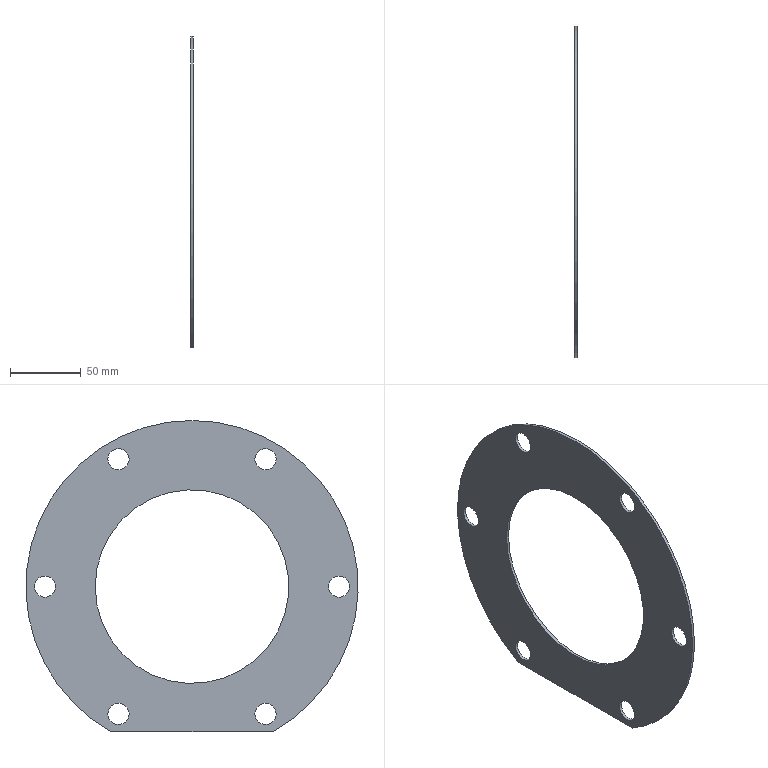Component | NX | T2_GASKET | 1 solid | 11 faces | box 2 x 235 x 220 mm | volume 52816 mm3 | cylinder 8 | plane 3 | commonest cylinder face diameters 15 x6 137 x1 235 x1
STEP:
#1=CARTESIAN_POINT('',(0.,0.,0.));
#2=DIRECTION('',(0.,0.,1.));
#3=DIRECTION('',(1.,0.,0.));
#4=AXIS2_PLACEMENT_3D('',#1,#2,#3);
#5=CARTESIAN_POINT('',(223.,-57.446,-105.5));
#6=VERTEX_POINT('',#5);
#7=CARTESIAN_POINT('',(223.,57.446,-105.5));
#8=VERTEX_POINT('',#7);
#9=CARTESIAN_POINT('',(223.,-57.446,-105.5));
#10=DIRECTION('',(0.,1.,0.));
#11=VECTOR('',#10,1.);
#12=LINE('',#9,#11);
#13=CARTESIAN_POINT('',(225.,-57.446,-105.5));
#14=DIRECTION('',(0.,0.,1.));
#15=DIRECTION('',(0.,1.,0.));
#16=AXIS2_PLACEMENT_3D('',#13,#14,#15);
#17=PLANE('',#16);
#18=CARTESIAN_POINT('',(0.,2.));
#19=DIRECTION('',(1.,0.));
#20=VECTOR('',#19,1.);
#21=LINE('',#18,#20);
#22=(GEOMETRIC_REPRESENTATION_CONTEXT(2)PARAMETRIC_REPRESENTATION_CONTEXT()REPRESENTATION_CONTEXT('',''));
#23=DEFINITIONAL_REPRESENTATION('',(#21),#22);
#24=PCURVE('',#17,#23);
#25=CARTESIAN_POINT('',(223.,0.,-3.));
#26=DIRECTION('',(1.,0.,0.));
#27=DIRECTION('',(0.,0.,-1.));
#28=AXIS2_PLACEMENT_3D('',#25,#26,#27);
#29=PLANE('',#28);
#30=CARTESIAN_POINT('',(102.5,-57.446));
#31=DIRECTION('',(0.,1.));
#32=VECTOR('',#31,1.);
#33=LINE('',#30,#32);
#34=(GEOMETRIC_REPRESENTATION_CONTEXT(2)PARAMETRIC_REPRESENTATION_CONTEXT()REPRESENTATION_CONTEXT('',''));
#35=DEFINITIONAL_REPRESENTATION('',(#33),#34);
#36=PCURVE('',#29,#35);
#37=SURFACE_CURVE('',#12,(#24,#36),.PCURVE_S1.);
#38=EDGE_CURVE('',#6,#8,#37,.T.);
#39=ORIENTED_EDGE('',*,*,#38,.T.);
#40=CARTESIAN_POINT('',(225.,57.446,-105.5));
#41=VERTEX_POINT('',#40);
#42=CARTESIAN_POINT('',(225.,57.446,-105.5));
#43=DIRECTION('',(-1.,0.,0.));
#44=VECTOR('',#43,1.);
#45=LINE('',#42,#44);
#46=CARTESIAN_POINT('',(114.891,0.));
#47=DIRECTION('',(0.,1.));
#48=VECTOR('',#47,1.);
#49=LINE('',#46,#48);
#50=(GEOMETRIC_REPRESENTATION_CONTEXT(2)PARAMETRIC_REPRESENTATION_CONTEXT()REPRESENTATION_CONTEXT('',''));
#51=DEFINITIONAL_REPRESENTATION('',(#49),#50);
#52=PCURVE('',#17,#51);
#53=CARTESIAN_POINT('',(225.,0.,-3.));
#54=DIRECTION('',(-1.,0.,0.));
#55=DIRECTION('',(0.,0.,1.));
#56=AXIS2_PLACEMENT_3D('',#53,#54,#55);
#57=CYLINDRICAL_SURFACE('',#56,117.5);
#58=CARTESIAN_POINT('',(2.631,0.));
#59=DIRECTION('',(0.,1.));
#60=VECTOR('',#59,1.);
#61=LINE('',#58,#60);
#62=(GEOMETRIC_REPRESENTATION_CONTEXT(2)PARAMETRIC_REPRESENTATION_CONTEXT()REPRESENTATION_CONTEXT('',''));
#63=DEFINITIONAL_REPRESENTATION('',(#61),#62);
#64=PCURVE('',#57,#63);
#65=SURFACE_CURVE('',#45,(#52,#64),.PCURVE_S1.);
#66=EDGE_CURVE('',#41,#8,#65,.T.);
#67=ORIENTED_EDGE('',*,*,#66,.F.);
#68=CARTESIAN_POINT('',(225.,-57.446,-105.5));
#69=VERTEX_POINT('',#68);
#70=CARTESIAN_POINT('',(225.,-57.446,-105.5));
#71=DIRECTION('',(0.,1.,0.));
#72=VECTOR('',#71,1.);
#73=LINE('',#70,#72);
#74=CARTESIAN_POINT('',(0.,0.));
#75=DIRECTION('',(1.,0.));
#76=VECTOR('',#75,1.);
#77=LINE('',#74,#76);
#78=(GEOMETRIC_REPRESENTATION_CONTEXT(2)PARAMETRIC_REPRESENTATION_CONTEXT()REPRESENTATION_CONTEXT('',''));
#79=DEFINITIONAL_REPRESENTATION('',(#77),#78);
#80=PCURVE('',#17,#79);
#81=CARTESIAN_POINT('',(225.,0.,-3.));
#82=DIRECTION('',(1.,0.,0.));
#83=DIRECTION('',(0.,0.,-1.));
#84=AXIS2_PLACEMENT_3D('',#81,#82,#83);
#85=PLANE('',#84);
#86=CARTESIAN_POINT('',(102.5,-57.446));
#87=DIRECTION('',(0.,1.));
#88=VECTOR('',#87,1.);
#89=LINE('',#86,#88);
#90=(GEOMETRIC_REPRESENTATION_CONTEXT(2)PARAMETRIC_REPRESENTATION_CONTEXT()REPRESENTATION_CONTEXT('',''));
#91=DEFINITIONAL_REPRESENTATION('',(#89),#90);
#92=PCURVE('',#85,#91);
#93=SURFACE_CURVE('',#73,(#80,#92),.PCURVE_S1.);
#94=EDGE_CURVE('',#69,#41,#93,.T.);
#95=ORIENTED_EDGE('',*,*,#94,.F.);
#96=CARTESIAN_POINT('',(225.,-57.446,-105.5));
#97=DIRECTION('',(1.,0.,0.));
#98=VECTOR('',#97,1.);
#99=LINE('',#96,#98);
#100=CARTESIAN_POINT('',(0.,0.));
#101=DIRECTION('',(0.,-1.));
#102=VECTOR('',#101,1.);
#103=LINE('',#100,#102);
#104=(GEOMETRIC_REPRESENTATION_CONTEXT(2)PARAMETRIC_REPRESENTATION_CONTEXT()REPRESENTATION_CONTEXT('',''));
#105=DEFINITIONAL_REPRESENTATION('',(#103),#104);
#106=PCURVE('',#17,#105);
#107=CARTESIAN_POINT('',(-2.631,0.));
#108=DIRECTION('',(0.,-1.));
#109=VECTOR('',#108,1.);
#110=LINE('',#107,#109);
#111=(GEOMETRIC_REPRESENTATION_CONTEXT(2)PARAMETRIC_REPRESENTATION_CONTEXT()REPRESENTATION_CONTEXT('',''));
#112=DEFINITIONAL_REPRESENTATION('',(#110),#111);
#113=PCURVE('',#57,#112);
#114=SURFACE_CURVE('',#99,(#106,#113),.PCURVE_S1.);
#115=EDGE_CURVE('',#6,#69,#114,.T.);
#116=ORIENTED_EDGE('',*,*,#115,.F.);
#117=EDGE_LOOP('',(#39,#67,#95,#116));
#118=FACE_BOUND('',#117,.T.);
#119=ADVANCED_FACE('',(#118),#17,.F.);
#120=CARTESIAN_POINT('',(225.,55.75,-99.562));
#121=VERTEX_POINT('',#120);
#122=CARTESIAN_POINT('',(225.,52.,-93.067));
#123=DIRECTION('',(1.,0.,0.));
#124=DIRECTION('',(0.,0.5,-0.866));
#125=AXIS2_PLACEMENT_3D('',#122,#123,#124);
#126=CIRCLE('',#125,7.5);
#127=CARTESIAN_POINT('',(225.,52.,-93.067));
#128=DIRECTION('',(-1.,0.,0.));
#129=DIRECTION('',(0.,0.,1.));
#130=AXIS2_PLACEMENT_3D('',#127,#128,#129);
#131=CYLINDRICAL_SURFACE('',#130,7.5);
#132=CARTESIAN_POINT('',(8.901,0.));
#133=DIRECTION('',(-1.,0.));
#134=VECTOR('',#133,1.);
#135=LINE('',#132,#134);
#136=(GEOMETRIC_REPRESENTATION_CONTEXT(2)PARAMETRIC_REPRESENTATION_CONTEXT()REPRESENTATION_CONTEXT('',''));
#137=DEFINITIONAL_REPRESENTATION('',(#135),#136);
#138=PCURVE('',#131,#137);
#139=CARTESIAN_POINT('',(90.067,52.));
#140=DIRECTION('',(0.866,0.5));
#141=AXIS2_PLACEMENT_2D('',#139,#140);
#142=CIRCLE('',#141,7.5);
#143=(GEOMETRIC_REPRESENTATION_CONTEXT(2)PARAMETRIC_REPRESENTATION_CONTEXT()REPRESENTATION_CONTEXT('',''));
#144=DEFINITIONAL_REPRESENTATION('',(#142),#143);
#145=PCURVE('',#85,#144);
#146=SURFACE_CURVE('',#126,(#138,#145),.PCURVE_S1.);
#147=EDGE_CURVE('',#121,#121,#146,.T.);
#148=ORIENTED_EDGE('',*,*,#147,.F.);
#149=CARTESIAN_POINT('',(223.,55.75,-99.562));
#150=VERTEX_POINT('',#149);
#151=CARTESIAN_POINT('',(225.,55.75,-99.562));
#152=CARTESIAN_POINT('',(223.,55.75,-99.562));
#153=B_SPLINE_CURVE_WITH_KNOTS('',1,(#151,#152),.UNSPECIFIED.,.F.,.F.,(2,2),(0.,2.),.PIECEWISE_BEZIER_KNOTS.);
#154=CARTESIAN_POINT('',(8.901,0.));
#155=DIRECTION('',(0.,1.));
#156=VECTOR('',#155,1.);
#157=LINE('',#154,#156);
#158=(GEOMETRIC_REPRESENTATION_CONTEXT(2)PARAMETRIC_REPRESENTATION_CONTEXT()REPRESENTATION_CONTEXT('',''));
#159=DEFINITIONAL_REPRESENTATION('',(#157),#158);
#160=PCURVE('',#131,#159);
#161=CARTESIAN_POINT('',(2.618,0.));
#162=DIRECTION('',(0.,1.));
#163=VECTOR('',#162,1.);
#164=LINE('',#161,#163);
#165=(GEOMETRIC_REPRESENTATION_CONTEXT(2)PARAMETRIC_REPRESENTATION_CONTEXT()REPRESENTATION_CONTEXT('',''));
#166=DEFINITIONAL_REPRESENTATION('',(#164),#165);
#167=PCURVE('',#131,#166);
#168=SEAM_CURVE('',#153,(#160,#167),.PCURVE_S1.);
#169=EDGE_CURVE('',#121,#150,#168,.T.);
#170=ORIENTED_EDGE('',*,*,#169,.T.);
#171=CARTESIAN_POINT('',(223.,52.,-93.067));
#172=DIRECTION('',(1.,0.,0.));
#173=DIRECTION('',(0.,0.5,-0.866));
#174=AXIS2_PLACEMENT_3D('',#171,#172,#173);
#175=CIRCLE('',#174,7.5);
#176=CARTESIAN_POINT('',(8.901,2.));
#177=DIRECTION('',(-1.,0.));
#178=VECTOR('',#177,1.);
#179=LINE('',#176,#178);
#180=(GEOMETRIC_REPRESENTATION_CONTEXT(2)PARAMETRIC_REPRESENTATION_CONTEXT()REPRESENTATION_CONTEXT('',''));
#181=DEFINITIONAL_REPRESENTATION('',(#179),#180);
#182=PCURVE('',#131,#181);
#183=CARTESIAN_POINT('',(90.067,52.));
#184=DIRECTION('',(0.866,0.5));
#185=AXIS2_PLACEMENT_2D('',#183,#184);
#186=CIRCLE('',#185,7.5);
#187=(GEOMETRIC_REPRESENTATION_CONTEXT(2)PARAMETRIC_REPRESENTATION_CONTEXT()REPRESENTATION_CONTEXT('',''));
#188=DEFINITIONAL_REPRESENTATION('',(#186),#187);
#189=PCURVE('',#29,#188);
#190=SURFACE_CURVE('',#175,(#182,#189),.PCURVE_S1.);
#191=EDGE_CURVE('',#150,#150,#190,.T.);
#192=ORIENTED_EDGE('',*,*,#191,.T.);
#193=ORIENTED_EDGE('',*,*,#169,.F.);
#194=EDGE_LOOP('',(#148,#170,#192,#193));
#195=FACE_BOUND('',#194,.F.);
#196=ADVANCED_FACE('',(#195),#131,.F.);
#197=CARTESIAN_POINT('',(225.,-55.75,-99.562));
#198=VERTEX_POINT('',#197);
#199=CARTESIAN_POINT('',(225.,-52.,-93.067));
#200=DIRECTION('',(1.,0.,0.));
#201=DIRECTION('',(0.,-0.5,-0.866));
#202=AXIS2_PLACEMENT_3D('',#199,#200,#201);
#203=CIRCLE('',#202,7.5);
#204=CARTESIAN_POINT('',(225.,-52.,-93.067));
#205=DIRECTION('',(-1.,0.,0.));
#206=DIRECTION('',(0.,0.,1.));
#207=AXIS2_PLACEMENT_3D('',#204,#205,#206);
#208=CYLINDRICAL_SURFACE('',#207,7.5);
#209=CARTESIAN_POINT('',(9.948,0.));
#210=DIRECTION('',(-1.,0.));
#211=VECTOR('',#210,1.);
#212=LINE('',#209,#211);
#213=(GEOMETRIC_REPRESENTATION_CONTEXT(2)PARAMETRIC_REPRESENTATION_CONTEXT()REPRESENTATION_CONTEXT('',''));
#214=DEFINITIONAL_REPRESENTATION('',(#212),#213);
#215=PCURVE('',#208,#214);
#216=CARTESIAN_POINT('',(90.067,-52.));
#217=DIRECTION('',(0.866,-0.5));
#218=AXIS2_PLACEMENT_2D('',#216,#217);
#219=CIRCLE('',#218,7.5);
#220=(GEOMETRIC_REPRESENTATION_CONTEXT(2)PARAMETRIC_REPRESENTATION_CONTEXT()REPRESENTATION_CONTEXT('',''));
#221=DEFINITIONAL_REPRESENTATION('',(#219),#220);
#222=PCURVE('',#85,#221);
#223=SURFACE_CURVE('',#203,(#215,#222),.PCURVE_S1.);
#224=EDGE_CURVE('',#198,#198,#223,.T.);
#225=ORIENTED_EDGE('',*,*,#224,.F.);
#226=CARTESIAN_POINT('',(223.,-55.75,-99.562));
#227=VERTEX_POINT('',#226);
#228=CARTESIAN_POINT('',(225.,-55.75,-99.562));
#229=CARTESIAN_POINT('',(223.,-55.75,-99.562));
#230=B_SPLINE_CURVE_WITH_KNOTS('',1,(#228,#229),.UNSPECIFIED.,.F.,.F.,(2,2),(0.,2.),.PIECEWISE_BEZIER_KNOTS.);
#231=CARTESIAN_POINT('',(9.948,0.));
#232=DIRECTION('',(0.,1.));
#233=VECTOR('',#232,1.);
#234=LINE('',#231,#233);
#235=(GEOMETRIC_REPRESENTATION_CONTEXT(2)PARAMETRIC_REPRESENTATION_CONTEXT()REPRESENTATION_CONTEXT('',''));
#236=DEFINITIONAL_REPRESENTATION('',(#234),#235);
#237=PCURVE('',#208,#236);
#238=CARTESIAN_POINT('',(3.665,0.));
#239=DIRECTION('',(0.,1.));
#240=VECTOR('',#239,1.);
#241=LINE('',#238,#240);
#242=(GEOMETRIC_REPRESENTATION_CONTEXT(2)PARAMETRIC_REPRESENTATION_CONTEXT()REPRESENTATION_CONTEXT('',''));
#243=DEFINITIONAL_REPRESENTATION('',(#241),#242);
#244=PCURVE('',#208,#243);
#245=SEAM_CURVE('',#230,(#237,#244),.PCURVE_S1.);
#246=EDGE_CURVE('',#198,#227,#245,.T.);
#247=ORIENTED_EDGE('',*,*,#246,.T.);
#248=CARTESIAN_POINT('',(223.,-52.,-93.067));
#249=DIRECTION('',(1.,0.,0.));
#250=DIRECTION('',(0.,-0.5,-0.866));
#251=AXIS2_PLACEMENT_3D('',#248,#249,#250);
#252=CIRCLE('',#251,7.5);
#253=CARTESIAN_POINT('',(9.948,2.));
#254=DIRECTION('',(-1.,0.));
#255=VECTOR('',#254,1.);
#256=LINE('',#253,#255);
#257=(GEOMETRIC_REPRESENTATION_CONTEXT(2)PARAMETRIC_REPRESENTATION_CONTEXT()REPRESENTATION_CONTEXT('',''));
#258=DEFINITIONAL_REPRESENTATION('',(#256),#257);
#259=PCURVE('',#208,#258);
#260=CARTESIAN_POINT('',(90.067,-52.));
#261=DIRECTION('',(0.866,-0.5));
#262=AXIS2_PLACEMENT_2D('',#260,#261);
#263=CIRCLE('',#262,7.5);
#264=(GEOMETRIC_REPRESENTATION_CONTEXT(2)PARAMETRIC_REPRESENTATION_CONTEXT()REPRESENTATION_CONTEXT('',''));
#265=DEFINITIONAL_REPRESENTATION('',(#263),#264);
#266=PCURVE('',#29,#265);
#267=SURFACE_CURVE('',#252,(#259,#266),.PCURVE_S1.);
#268=EDGE_CURVE('',#227,#227,#267,.T.);
#269=ORIENTED_EDGE('',*,*,#268,.T.);
#270=ORIENTED_EDGE('',*,*,#246,.F.);
#271=EDGE_LOOP('',(#225,#247,#269,#270));
#272=FACE_BOUND('',#271,.F.);
#273=ADVANCED_FACE('',(#272),#208,.F.);
#274=CARTESIAN_POINT('',(225.,-111.5,-3.));
#275=VERTEX_POINT('',#274);
#276=CARTESIAN_POINT('',(225.,-104.,-3.));
#277=DIRECTION('',(1.,0.,0.));
#278=DIRECTION('',(0.,-1.,0.));
#279=AXIS2_PLACEMENT_3D('',#276,#277,#278);
#280=CIRCLE('',#279,7.5);
#281=CARTESIAN_POINT('',(225.,-104.,-3.));
#282=DIRECTION('',(-1.,0.,0.));
#283=DIRECTION('',(0.,0.,1.));
#284=AXIS2_PLACEMENT_3D('',#281,#282,#283);
#285=CYLINDRICAL_SURFACE('',#284,7.5);
#286=CARTESIAN_POINT('',(10.996,0.));
#287=DIRECTION('',(-1.,0.));
#288=VECTOR('',#287,1.);
#289=LINE('',#286,#288);
#290=(GEOMETRIC_REPRESENTATION_CONTEXT(2)PARAMETRIC_REPRESENTATION_CONTEXT()REPRESENTATION_CONTEXT('',''));
#291=DEFINITIONAL_REPRESENTATION('',(#289),#290);
#292=PCURVE('',#285,#291);
#293=CARTESIAN_POINT('',(0.,-104.));
#294=DIRECTION('',(-0.,-1.));
#295=AXIS2_PLACEMENT_2D('',#293,#294);
#296=CIRCLE('',#295,7.5);
#297=(GEOMETRIC_REPRESENTATION_CONTEXT(2)PARAMETRIC_REPRESENTATION_CONTEXT()REPRESENTATION_CONTEXT('',''));
#298=DEFINITIONAL_REPRESENTATION('',(#296),#297);
#299=PCURVE('',#85,#298);
#300=SURFACE_CURVE('',#280,(#292,#299),.PCURVE_S1.);
#301=EDGE_CURVE('',#275,#275,#300,.T.);
#302=ORIENTED_EDGE('',*,*,#301,.F.);
#303=CARTESIAN_POINT('',(223.,-111.5,-3.));
#304=VERTEX_POINT('',#303);
#305=CARTESIAN_POINT('',(225.,-111.5,-3.));
#306=CARTESIAN_POINT('',(223.,-111.5,-3.));
#307=B_SPLINE_CURVE_WITH_KNOTS('',1,(#305,#306),.UNSPECIFIED.,.F.,.F.,(2,2),(0.,2.),.PIECEWISE_BEZIER_KNOTS.);
#308=CARTESIAN_POINT('',(10.996,0.));
#309=DIRECTION('',(0.,1.));
#310=VECTOR('',#309,1.);
#311=LINE('',#308,#310);
#312=(GEOMETRIC_REPRESENTATION_CONTEXT(2)PARAMETRIC_REPRESENTATION_CONTEXT()REPRESENTATION_CONTEXT('',''));
#313=DEFINITIONAL_REPRESENTATION('',(#311),#312);
#314=PCURVE('',#285,#313);
#315=CARTESIAN_POINT('',(4.712,0.));
#316=DIRECTION('',(0.,1.));
#317=VECTOR('',#316,1.);
#318=LINE('',#315,#317);
#319=(GEOMETRIC_REPRESENTATION_CONTEXT(2)PARAMETRIC_REPRESENTATION_CONTEXT()REPRESENTATION_CONTEXT('',''));
#320=DEFINITIONAL_REPRESENTATION('',(#318),#319);
#321=PCURVE('',#285,#320);
#322=SEAM_CURVE('',#307,(#314,#321),.PCURVE_S1.);
#323=EDGE_CURVE('',#275,#304,#322,.T.);
#324=ORIENTED_EDGE('',*,*,#323,.T.);
#325=CARTESIAN_POINT('',(223.,-104.,-3.));
#326=DIRECTION('',(1.,0.,0.));
#327=DIRECTION('',(0.,-1.,0.));
#328=AXIS2_PLACEMENT_3D('',#325,#326,#327);
#329=CIRCLE('',#328,7.5);
#330=CARTESIAN_POINT('',(10.996,2.));
#331=DIRECTION('',(-1.,0.));
#332=VECTOR('',#331,1.);
#333=LINE('',#330,#332);
#334=(GEOMETRIC_REPRESENTATION_CONTEXT(2)PARAMETRIC_REPRESENTATION_CONTEXT()REPRESENTATION_CONTEXT('',''));
#335=DEFINITIONAL_REPRESENTATION('',(#333),#334);
#336=PCURVE('',#285,#335);
#337=CARTESIAN_POINT('',(0.,-104.));
#338=DIRECTION('',(-0.,-1.));
#339=AXIS2_PLACEMENT_2D('',#337,#338);
#340=CIRCLE('',#339,7.5);
#341=(GEOMETRIC_REPRESENTATION_CONTEXT(2)PARAMETRIC_REPRESENTATION_CONTEXT()REPRESENTATION_CONTEXT('',''));
#342=DEFINITIONAL_REPRESENTATION('',(#340),#341);
#343=PCURVE('',#29,#342);
#344=SURFACE_CURVE('',#329,(#336,#343),.PCURVE_S1.);
#345=EDGE_CURVE('',#304,#304,#344,.T.);
#346=ORIENTED_EDGE('',*,*,#345,.T.);
#347=ORIENTED_EDGE('',*,*,#323,.F.);
#348=EDGE_LOOP('',(#302,#324,#346,#347));
#349=FACE_BOUND('',#348,.F.);
#350=ADVANCED_FACE('',(#349),#285,.F.);
#351=CARTESIAN_POINT('',(225.,68.5,-3.));
#352=VERTEX_POINT('',#351);
#353=CARTESIAN_POINT('',(225.,0.,-3.));
#354=DIRECTION('',(1.,0.,0.));
#355=DIRECTION('',(0.,1.,-0.));
#356=AXIS2_PLACEMENT_3D('',#353,#354,#355);
#357=CIRCLE('',#356,68.5);
#358=CARTESIAN_POINT('',(225.,0.,-3.));
#359=DIRECTION('',(-1.,0.,0.));
#360=DIRECTION('',(0.,0.,1.));
#361=AXIS2_PLACEMENT_3D('',#358,#359,#360);
#362=CYLINDRICAL_SURFACE('',#361,68.5);
#363=CARTESIAN_POINT('',(7.854,0.));
#364=DIRECTION('',(-1.,0.));
#365=VECTOR('',#364,1.);
#366=LINE('',#363,#365);
#367=(GEOMETRIC_REPRESENTATION_CONTEXT(2)PARAMETRIC_REPRESENTATION_CONTEXT()REPRESENTATION_CONTEXT('',''));
#368=DEFINITIONAL_REPRESENTATION('',(#366),#367);
#369=PCURVE('',#362,#368);
#370=CARTESIAN_POINT('',(0.,0.));
#371=DIRECTION('',(0.,1.));
#372=AXIS2_PLACEMENT_2D('',#370,#371);
#373=CIRCLE('',#372,68.5);
#374=(GEOMETRIC_REPRESENTATION_CONTEXT(2)PARAMETRIC_REPRESENTATION_CONTEXT()REPRESENTATION_CONTEXT('',''));
#375=DEFINITIONAL_REPRESENTATION('',(#373),#374);
#376=PCURVE('',#85,#375);
#377=SURFACE_CURVE('',#357,(#369,#376),.PCURVE_S1.);
#378=EDGE_CURVE('',#352,#352,#377,.T.);
#379=ORIENTED_EDGE('',*,*,#378,.F.);
#380=CARTESIAN_POINT('',(223.,68.5,-3.));
#381=VERTEX_POINT('',#380);
#382=CARTESIAN_POINT('',(225.,68.5,-3.));
#383=CARTESIAN_POINT('',(223.,68.5,-3.));
#384=B_SPLINE_CURVE_WITH_KNOTS('',1,(#382,#383),.UNSPECIFIED.,.F.,.F.,(2,2),(0.,2.),.PIECEWISE_BEZIER_KNOTS.);
#385=CARTESIAN_POINT('',(7.854,0.));
#386=DIRECTION('',(0.,1.));
#387=VECTOR('',#386,1.);
#388=LINE('',#385,#387);
#389=(GEOMETRIC_REPRESENTATION_CONTEXT(2)PARAMETRIC_REPRESENTATION_CONTEXT()REPRESENTATION_CONTEXT('',''));
#390=DEFINITIONAL_REPRESENTATION('',(#388),#389);
#391=PCURVE('',#362,#390);
#392=CARTESIAN_POINT('',(1.571,0.));
#393=DIRECTION('',(0.,1.));
#394=VECTOR('',#393,1.);
#395=LINE('',#392,#394);
#396=(GEOMETRIC_REPRESENTATION_CONTEXT(2)PARAMETRIC_REPRESENTATION_CONTEXT()REPRESENTATION_CONTEXT('',''));
#397=DEFINITIONAL_REPRESENTATION('',(#395),#396);
#398=PCURVE('',#362,#397);
#399=SEAM_CURVE('',#384,(#391,#398),.PCURVE_S1.);
#400=EDGE_CURVE('',#352,#381,#399,.T.);
#401=ORIENTED_EDGE('',*,*,#400,.T.);
#402=CARTESIAN_POINT('',(223.,0.,-3.));
#403=DIRECTION('',(1.,0.,0.));
#404=DIRECTION('',(0.,1.,-0.));
#405=AXIS2_PLACEMENT_3D('',#402,#403,#404);
#406=CIRCLE('',#405,68.5);
#407=CARTESIAN_POINT('',(7.854,2.));
#408=DIRECTION('',(-1.,0.));
#409=VECTOR('',#408,1.);
#410=LINE('',#407,#409);
#411=(GEOMETRIC_REPRESENTATION_CONTEXT(2)PARAMETRIC_REPRESENTATION_CONTEXT()REPRESENTATION_CONTEXT('',''));
#412=DEFINITIONAL_REPRESENTATION('',(#410),#411);
#413=PCURVE('',#362,#412);
#414=CARTESIAN_POINT('',(0.,0.));
#415=DIRECTION('',(0.,1.));
#416=AXIS2_PLACEMENT_2D('',#414,#415);
#417=CIRCLE('',#416,68.5);
#418=(GEOMETRIC_REPRESENTATION_CONTEXT(2)PARAMETRIC_REPRESENTATION_CONTEXT()REPRESENTATION_CONTEXT('',''));
#419=DEFINITIONAL_REPRESENTATION('',(#417),#418);
#420=PCURVE('',#29,#419);
#421=SURFACE_CURVE('',#406,(#413,#420),.PCURVE_S1.);
#422=EDGE_CURVE('',#381,#381,#421,.T.);
#423=ORIENTED_EDGE('',*,*,#422,.T.);
#424=ORIENTED_EDGE('',*,*,#400,.F.);
#425=EDGE_LOOP('',(#379,#401,#423,#424));
#426=FACE_BOUND('',#425,.F.);
#427=ADVANCED_FACE('',(#426),#362,.F.);
#428=CARTESIAN_POINT('',(225.,-55.75,93.562));
#429=VERTEX_POINT('',#428);
#430=CARTESIAN_POINT('',(225.,-52.,87.067));
#431=DIRECTION('',(1.,0.,0.));
#432=DIRECTION('',(0.,-0.5,0.866));
#433=AXIS2_PLACEMENT_3D('',#430,#431,#432);
#434=CIRCLE('',#433,7.5);
#435=CARTESIAN_POINT('',(225.,-52.,87.067));
#436=DIRECTION('',(-1.,0.,0.));
#437=DIRECTION('',(0.,0.,1.));
#438=AXIS2_PLACEMENT_3D('',#435,#436,#437);
#439=CYLINDRICAL_SURFACE('',#438,7.5);
#440=CARTESIAN_POINT('',(12.043,0.));
#441=DIRECTION('',(-1.,0.));
#442=VECTOR('',#441,1.);
#443=LINE('',#440,#442);
#444=(GEOMETRIC_REPRESENTATION_CONTEXT(2)PARAMETRIC_REPRESENTATION_CONTEXT()REPRESENTATION_CONTEXT('',''));
#445=DEFINITIONAL_REPRESENTATION('',(#443),#444);
#446=PCURVE('',#439,#445);
#447=CARTESIAN_POINT('',(-90.067,-52.));
#448=DIRECTION('',(-0.866,-0.5));
#449=AXIS2_PLACEMENT_2D('',#447,#448);
#450=CIRCLE('',#449,7.5);
#451=(GEOMETRIC_REPRESENTATION_CONTEXT(2)PARAMETRIC_REPRESENTATION_CONTEXT()REPRESENTATION_CONTEXT('',''));
#452=DEFINITIONAL_REPRESENTATION('',(#450),#451);
#453=PCURVE('',#85,#452);
#454=SURFACE_CURVE('',#434,(#446,#453),.PCURVE_S1.);
#455=EDGE_CURVE('',#429,#429,#454,.T.);
#456=ORIENTED_EDGE('',*,*,#455,.F.);
#457=CARTESIAN_POINT('',(223.,-55.75,93.562));
#458=VERTEX_POINT('',#457);
#459=CARTESIAN_POINT('',(225.,-55.75,93.562));
#460=CARTESIAN_POINT('',(223.,-55.75,93.562));
#461=B_SPLINE_CURVE_WITH_KNOTS('',1,(#459,#460),.UNSPECIFIED.,.F.,.F.,(2,2),(0.,2.),.PIECEWISE_BEZIER_KNOTS.);
#462=CARTESIAN_POINT('',(12.043,0.));
#463=DIRECTION('',(0.,1.));
#464=VECTOR('',#463,1.);
#465=LINE('',#462,#464);
#466=(GEOMETRIC_REPRESENTATION_CONTEXT(2)PARAMETRIC_REPRESENTATION_CONTEXT()REPRESENTATION_CONTEXT('',''));
#467=DEFINITIONAL_REPRESENTATION('',(#465),#466);
#468=PCURVE('',#439,#467);
#469=CARTESIAN_POINT('',(5.76,0.));
#470=DIRECTION('',(0.,1.));
#471=VECTOR('',#470,1.);
#472=LINE('',#469,#471);
#473=(GEOMETRIC_REPRESENTATION_CONTEXT(2)PARAMETRIC_REPRESENTATION_CONTEXT()REPRESENTATION_CONTEXT('',''));
#474=DEFINITIONAL_REPRESENTATION('',(#472),#473);
#475=PCURVE('',#439,#474);
#476=SEAM_CURVE('',#461,(#468,#475),.PCURVE_S1.);
#477=EDGE_CURVE('',#429,#458,#476,.T.);
#478=ORIENTED_EDGE('',*,*,#477,.T.);
#479=CARTESIAN_POINT('',(223.,-52.,87.067));
#480=DIRECTION('',(1.,0.,0.));
#481=DIRECTION('',(0.,-0.5,0.866));
#482=AXIS2_PLACEMENT_3D('',#479,#480,#481);
#483=CIRCLE('',#482,7.5);
#484=CARTESIAN_POINT('',(12.043,2.));
#485=DIRECTION('',(-1.,0.));
#486=VECTOR('',#485,1.);
#487=LINE('',#484,#486);
#488=(GEOMETRIC_REPRESENTATION_CONTEXT(2)PARAMETRIC_REPRESENTATION_CONTEXT()REPRESENTATION_CONTEXT('',''));
#489=DEFINITIONAL_REPRESENTATION('',(#487),#488);
#490=PCURVE('',#439,#489);
#491=CARTESIAN_POINT('',(-90.067,-52.));
#492=DIRECTION('',(-0.866,-0.5));
#493=AXIS2_PLACEMENT_2D('',#491,#492);
#494=CIRCLE('',#493,7.5);
#495=(GEOMETRIC_REPRESENTATION_CONTEXT(2)PARAMETRIC_REPRESENTATION_CONTEXT()REPRESENTATION_CONTEXT('',''));
#496=DEFINITIONAL_REPRESENTATION('',(#494),#495);
#497=PCURVE('',#29,#496);
#498=SURFACE_CURVE('',#483,(#490,#497),.PCURVE_S1.);
#499=EDGE_CURVE('',#458,#458,#498,.T.);
#500=ORIENTED_EDGE('',*,*,#499,.T.);
#501=ORIENTED_EDGE('',*,*,#477,.F.);
#502=EDGE_LOOP('',(#456,#478,#500,#501));
#503=FACE_BOUND('',#502,.F.);
#504=ADVANCED_FACE('',(#503),#439,.F.);
#505=CARTESIAN_POINT('',(225.,55.75,93.562));
#506=VERTEX_POINT('',#505);
#507=CARTESIAN_POINT('',(225.,52.,87.067));
#508=DIRECTION('',(1.,0.,0.));
#509=DIRECTION('',(0.,0.5,0.866));
#510=AXIS2_PLACEMENT_3D('',#507,#508,#509);
#511=CIRCLE('',#510,7.5);
#512=CARTESIAN_POINT('',(225.,52.,87.067));
#513=DIRECTION('',(-1.,0.,0.));
#514=DIRECTION('',(0.,0.,1.));
#515=AXIS2_PLACEMENT_3D('',#512,#513,#514);
#516=CYLINDRICAL_SURFACE('',#515,7.5);
#517=CARTESIAN_POINT('',(6.807,0.));
#518=DIRECTION('',(-1.,0.));
#519=VECTOR('',#518,1.);
#520=LINE('',#517,#519);
#521=(GEOMETRIC_REPRESENTATION_CONTEXT(2)PARAMETRIC_REPRESENTATION_CONTEXT()REPRESENTATION_CONTEXT('',''));
#522=DEFINITIONAL_REPRESENTATION('',(#520),#521);
#523=PCURVE('',#516,#522);
#524=CARTESIAN_POINT('',(-90.067,52.));
#525=DIRECTION('',(-0.866,0.5));
#526=AXIS2_PLACEMENT_2D('',#524,#525);
#527=CIRCLE('',#526,7.5);
#528=(GEOMETRIC_REPRESENTATION_CONTEXT(2)PARAMETRIC_REPRESENTATION_CONTEXT()REPRESENTATION_CONTEXT('',''));
#529=DEFINITIONAL_REPRESENTATION('',(#527),#528);
#530=PCURVE('',#85,#529);
#531=SURFACE_CURVE('',#511,(#523,#530),.PCURVE_S1.);
#532=EDGE_CURVE('',#506,#506,#531,.T.);
#533=ORIENTED_EDGE('',*,*,#532,.F.);
#534=CARTESIAN_POINT('',(223.,55.75,93.562));
#535=VERTEX_POINT('',#534);
#536=CARTESIAN_POINT('',(225.,55.75,93.562));
#537=CARTESIAN_POINT('',(223.,55.75,93.562));
#538=B_SPLINE_CURVE_WITH_KNOTS('',1,(#536,#537),.UNSPECIFIED.,.F.,.F.,(2,2),(0.,2.),.PIECEWISE_BEZIER_KNOTS.);
#539=CARTESIAN_POINT('',(6.807,0.));
#540=DIRECTION('',(0.,1.));
#541=VECTOR('',#540,1.);
#542=LINE('',#539,#541);
#543=(GEOMETRIC_REPRESENTATION_CONTEXT(2)PARAMETRIC_REPRESENTATION_CONTEXT()REPRESENTATION_CONTEXT('',''));
#544=DEFINITIONAL_REPRESENTATION('',(#542),#543);
#545=PCURVE('',#516,#544);
#546=CARTESIAN_POINT('',(0.5236,0.));
#547=DIRECTION('',(0.,1.));
#548=VECTOR('',#547,1.);
#549=LINE('',#546,#548);
#550=(GEOMETRIC_REPRESENTATION_CONTEXT(2)PARAMETRIC_REPRESENTATION_CONTEXT()REPRESENTATION_CONTEXT('',''));
#551=DEFINITIONAL_REPRESENTATION('',(#549),#550);
#552=PCURVE('',#516,#551);
#553=SEAM_CURVE('',#538,(#545,#552),.PCURVE_S1.);
#554=EDGE_CURVE('',#506,#535,#553,.T.);
#555=ORIENTED_EDGE('',*,*,#554,.T.);
#556=CARTESIAN_POINT('',(223.,52.,87.067));
#557=DIRECTION('',(1.,0.,0.));
#558=DIRECTION('',(0.,0.5,0.866));
#559=AXIS2_PLACEMENT_3D('',#556,#557,#558);
#560=CIRCLE('',#559,7.5);
#561=CARTESIAN_POINT('',(6.807,2.));
#562=DIRECTION('',(-1.,0.));
#563=VECTOR('',#562,1.);
#564=LINE('',#561,#563);
#565=(GEOMETRIC_REPRESENTATION_CONTEXT(2)PARAMETRIC_REPRESENTATION_CONTEXT()REPRESENTATION_CONTEXT('',''));
#566=DEFINITIONAL_REPRESENTATION('',(#564),#565);
#567=PCURVE('',#516,#566);
#568=CARTESIAN_POINT('',(-90.067,52.));
#569=DIRECTION('',(-0.866,0.5));
#570=AXIS2_PLACEMENT_2D('',#568,#569);
#571=CIRCLE('',#570,7.5);
#572=(GEOMETRIC_REPRESENTATION_CONTEXT(2)PARAMETRIC_REPRESENTATION_CONTEXT()REPRESENTATION_CONTEXT('',''));
#573=DEFINITIONAL_REPRESENTATION('',(#571),#572);
#574=PCURVE('',#29,#573);
#575=SURFACE_CURVE('',#560,(#567,#574),.PCURVE_S1.);
#576=EDGE_CURVE('',#535,#535,#575,.T.);
#577=ORIENTED_EDGE('',*,*,#576,.T.);
#578=ORIENTED_EDGE('',*,*,#554,.F.);
#579=EDGE_LOOP('',(#533,#555,#577,#578));
#580=FACE_BOUND('',#579,.F.);
#581=ADVANCED_FACE('',(#580),#516,.F.);
#582=CARTESIAN_POINT('',(223.,0.,-3.));
#583=DIRECTION('',(1.,0.,0.));
#584=DIRECTION('',(0.,1.,-0.));
#585=AXIS2_PLACEMENT_3D('',#582,#583,#584);
#586=CIRCLE('',#585,117.5);
#587=CARTESIAN_POINT('',(7.854,2.));
#588=DIRECTION('',(-1.,0.));
#589=VECTOR('',#588,1.);
#590=LINE('',#587,#589);
#591=(GEOMETRIC_REPRESENTATION_CONTEXT(2)PARAMETRIC_REPRESENTATION_CONTEXT()REPRESENTATION_CONTEXT('',''));
#592=DEFINITIONAL_REPRESENTATION('',(#590),#591);
#593=PCURVE('',#57,#592);
#594=CARTESIAN_POINT('',(0.,0.));
#595=DIRECTION('',(0.,1.));
#596=AXIS2_PLACEMENT_2D('',#594,#595);
#597=CIRCLE('',#596,117.5);
#598=(GEOMETRIC_REPRESENTATION_CONTEXT(2)PARAMETRIC_REPRESENTATION_CONTEXT()REPRESENTATION_CONTEXT('',''));
#599=DEFINITIONAL_REPRESENTATION('',(#597),#598);
#600=PCURVE('',#29,#599);
#601=SURFACE_CURVE('',#586,(#593,#600),.PCURVE_S1.);
#602=EDGE_CURVE('',#8,#6,#601,.T.);
#603=ORIENTED_EDGE('',*,*,#602,.T.);
#604=ORIENTED_EDGE('',*,*,#115,.T.);
#605=CARTESIAN_POINT('',(225.,0.,-3.));
#606=DIRECTION('',(1.,0.,0.));
#607=DIRECTION('',(0.,1.,-0.));
#608=AXIS2_PLACEMENT_3D('',#605,#606,#607);
#609=CIRCLE('',#608,117.5);
#610=CARTESIAN_POINT('',(7.854,0.));
#611=DIRECTION('',(-1.,0.));
#612=VECTOR('',#611,1.);
#613=LINE('',#610,#612);
#614=(GEOMETRIC_REPRESENTATION_CONTEXT(2)PARAMETRIC_REPRESENTATION_CONTEXT()REPRESENTATION_CONTEXT('',''));
#615=DEFINITIONAL_REPRESENTATION('',(#613),#614);
#616=PCURVE('',#57,#615);
#617=CARTESIAN_POINT('',(0.,0.));
#618=DIRECTION('',(0.,1.));
#619=AXIS2_PLACEMENT_2D('',#617,#618);
#620=CIRCLE('',#619,117.5);
#621=(GEOMETRIC_REPRESENTATION_CONTEXT(2)PARAMETRIC_REPRESENTATION_CONTEXT()REPRESENTATION_CONTEXT('',''));
#622=DEFINITIONAL_REPRESENTATION('',(#620),#621);
#623=PCURVE('',#85,#622);
#624=SURFACE_CURVE('',#609,(#616,#623),.PCURVE_S1.);
#625=EDGE_CURVE('',#41,#69,#624,.T.);
#626=ORIENTED_EDGE('',*,*,#625,.F.);
#627=ORIENTED_EDGE('',*,*,#66,.T.);
#628=EDGE_LOOP('',(#603,#604,#626,#627));
#629=FACE_BOUND('',#628,.T.);
#630=ADVANCED_FACE('',(#629),#57,.T.);
#631=CARTESIAN_POINT('',(225.,111.5,-3.));
#632=VERTEX_POINT('',#631);
#633=CARTESIAN_POINT('',(225.,104.,-3.));
#634=DIRECTION('',(1.,0.,0.));
#635=DIRECTION('',(0.,1.,-0.));
#636=AXIS2_PLACEMENT_3D('',#633,#634,#635);
#637=CIRCLE('',#636,7.5);
#638=CARTESIAN_POINT('',(225.,104.,-3.));
#639=DIRECTION('',(-1.,0.,0.));
#640=DIRECTION('',(0.,0.,1.));
#641=AXIS2_PLACEMENT_3D('',#638,#639,#640);
#642=CYLINDRICAL_SURFACE('',#641,7.5);
#643=CARTESIAN_POINT('',(7.854,0.));
#644=DIRECTION('',(-1.,0.));
#645=VECTOR('',#644,1.);
#646=LINE('',#643,#645);
#647=(GEOMETRIC_REPRESENTATION_CONTEXT(2)PARAMETRIC_REPRESENTATION_CONTEXT()REPRESENTATION_CONTEXT('',''));
#648=DEFINITIONAL_REPRESENTATION('',(#646),#647);
#649=PCURVE('',#642,#648);
#650=CARTESIAN_POINT('',(0.,104.));
#651=DIRECTION('',(0.,1.));
#652=AXIS2_PLACEMENT_2D('',#650,#651);
#653=CIRCLE('',#652,7.5);
#654=(GEOMETRIC_REPRESENTATION_CONTEXT(2)PARAMETRIC_REPRESENTATION_CONTEXT()REPRESENTATION_CONTEXT('',''));
#655=DEFINITIONAL_REPRESENTATION('',(#653),#654);
#656=PCURVE('',#85,#655);
#657=SURFACE_CURVE('',#637,(#649,#656),.PCURVE_S1.);
#658=EDGE_CURVE('',#632,#632,#657,.T.);
#659=ORIENTED_EDGE('',*,*,#658,.F.);
#660=CARTESIAN_POINT('',(223.,111.5,-3.));
#661=VERTEX_POINT('',#660);
#662=CARTESIAN_POINT('',(225.,111.5,-3.));
#663=CARTESIAN_POINT('',(223.,111.5,-3.));
#664=B_SPLINE_CURVE_WITH_KNOTS('',1,(#662,#663),.UNSPECIFIED.,.F.,.F.,(2,2),(0.,2.),.PIECEWISE_BEZIER_KNOTS.);
#665=CARTESIAN_POINT('',(7.854,0.));
#666=DIRECTION('',(0.,1.));
#667=VECTOR('',#666,1.);
#668=LINE('',#665,#667);
#669=(GEOMETRIC_REPRESENTATION_CONTEXT(2)PARAMETRIC_REPRESENTATION_CONTEXT()REPRESENTATION_CONTEXT('',''));
#670=DEFINITIONAL_REPRESENTATION('',(#668),#669);
#671=PCURVE('',#642,#670);
#672=CARTESIAN_POINT('',(1.571,0.));
#673=DIRECTION('',(0.,1.));
#674=VECTOR('',#673,1.);
#675=LINE('',#672,#674);
#676=(GEOMETRIC_REPRESENTATION_CONTEXT(2)PARAMETRIC_REPRESENTATION_CONTEXT()REPRESENTATION_CONTEXT('',''));
#677=DEFINITIONAL_REPRESENTATION('',(#675),#676);
#678=PCURVE('',#642,#677);
#679=SEAM_CURVE('',#664,(#671,#678),.PCURVE_S1.);
#680=EDGE_CURVE('',#632,#661,#679,.T.);
#681=ORIENTED_EDGE('',*,*,#680,.T.);
#682=CARTESIAN_POINT('',(223.,104.,-3.));
#683=DIRECTION('',(1.,0.,0.));
#684=DIRECTION('',(0.,1.,-0.));
#685=AXIS2_PLACEMENT_3D('',#682,#683,#684);
#686=CIRCLE('',#685,7.5);
#687=CARTESIAN_POINT('',(7.854,2.));
#688=DIRECTION('',(-1.,0.));
#689=VECTOR('',#688,1.);
#690=LINE('',#687,#689);
#691=(GEOMETRIC_REPRESENTATION_CONTEXT(2)PARAMETRIC_REPRESENTATION_CONTEXT()REPRESENTATION_CONTEXT('',''));
#692=DEFINITIONAL_REPRESENTATION('',(#690),#691);
#693=PCURVE('',#642,#692);
#694=CARTESIAN_POINT('',(0.,104.));
#695=DIRECTION('',(0.,1.));
#696=AXIS2_PLACEMENT_2D('',#694,#695);
#697=CIRCLE('',#696,7.5);
#698=(GEOMETRIC_REPRESENTATION_CONTEXT(2)PARAMETRIC_REPRESENTATION_CONTEXT()REPRESENTATION_CONTEXT('',''));
#699=DEFINITIONAL_REPRESENTATION('',(#697),#698);
#700=PCURVE('',#29,#699);
#701=SURFACE_CURVE('',#686,(#693,#700),.PCURVE_S1.);
#702=EDGE_CURVE('',#661,#661,#701,.T.);
#703=ORIENTED_EDGE('',*,*,#702,.T.);
#704=ORIENTED_EDGE('',*,*,#680,.F.);
#705=EDGE_LOOP('',(#659,#681,#703,#704));
#706=FACE_BOUND('',#705,.F.);
#707=ADVANCED_FACE('',(#706),#642,.F.);
#708=ORIENTED_EDGE('',*,*,#94,.T.);
#709=ORIENTED_EDGE('',*,*,#625,.T.);
#710=EDGE_LOOP('',(#708,#709));
#711=FACE_BOUND('',#710,.T.);
#712=ORIENTED_EDGE('',*,*,#532,.F.);
#713=EDGE_LOOP('',(#712));
#714=FACE_BOUND('',#713,.T.);
#715=ORIENTED_EDGE('',*,*,#455,.F.);
#716=EDGE_LOOP('',(#715));
#717=FACE_BOUND('',#716,.T.);
#718=ORIENTED_EDGE('',*,*,#378,.F.);
#719=EDGE_LOOP('',(#718));
#720=FACE_BOUND('',#719,.T.);
#721=ORIENTED_EDGE('',*,*,#301,.F.);
#722=EDGE_LOOP('',(#721));
#723=FACE_BOUND('',#722,.T.);
#724=ORIENTED_EDGE('',*,*,#224,.F.);
#725=EDGE_LOOP('',(#724));
#726=FACE_BOUND('',#725,.T.);
#727=ORIENTED_EDGE('',*,*,#147,.F.);
#728=EDGE_LOOP('',(#727));
#729=FACE_BOUND('',#728,.T.);
#730=ORIENTED_EDGE('',*,*,#658,.F.);
#731=EDGE_LOOP('',(#730));
#732=FACE_BOUND('',#731,.T.);
#733=ADVANCED_FACE('',(#711,#714,#717,#720,#723,#726,#729,#732),#85,.T.);
#734=ORIENTED_EDGE('',*,*,#38,.F.);
#735=ORIENTED_EDGE('',*,*,#602,.F.);
#736=EDGE_LOOP('',(#734,#735));
#737=FACE_BOUND('',#736,.T.);
#738=ORIENTED_EDGE('',*,*,#576,.T.);
#739=EDGE_LOOP('',(#738));
#740=FACE_BOUND('',#739,.T.);
#741=ORIENTED_EDGE('',*,*,#499,.T.);
#742=EDGE_LOOP('',(#741));
#743=FACE_BOUND('',#742,.T.);
#744=ORIENTED_EDGE('',*,*,#422,.T.);
#745=EDGE_LOOP('',(#744));
#746=FACE_BOUND('',#745,.T.);
#747=ORIENTED_EDGE('',*,*,#345,.T.);
#748=EDGE_LOOP('',(#747));
#749=FACE_BOUND('',#748,.T.);
#750=ORIENTED_EDGE('',*,*,#268,.T.);
#751=EDGE_LOOP('',(#750));
#752=FACE_BOUND('',#751,.T.);
#753=ORIENTED_EDGE('',*,*,#191,.T.);
#754=EDGE_LOOP('',(#753));
#755=FACE_BOUND('',#754,.T.);
#756=ORIENTED_EDGE('',*,*,#702,.T.);
#757=EDGE_LOOP('',(#756));
#758=FACE_BOUND('',#757,.T.);
#759=ADVANCED_FACE('',(#737,#740,#743,#746,#749,#752,#755,#758),#29,.F.);
#760=CLOSED_SHELL('',(#119,#196,#273,#350,#427,#504,#581,#630,#707,#733,#759));
#761=MANIFOLD_SOLID_BREP('',#760);
#762=(LENGTH_UNIT()NAMED_UNIT(*)SI_UNIT(.MILLI.,.METRE.));
#763=UNCERTAINTY_MEASURE_WITH_UNIT(LENGTH_MEASURE(0.000005),#762,'','');
#764=(NAMED_UNIT(*)PLANE_ANGLE_UNIT()SI_UNIT($,.RADIAN.));
#765=(NAMED_UNIT(*)SI_UNIT($,.STERADIAN.)SOLID_ANGLE_UNIT());
#766=(GEOMETRIC_REPRESENTATION_CONTEXT(3)GLOBAL_UNCERTAINTY_ASSIGNED_CONTEXT((#763))GLOBAL_UNIT_ASSIGNED_CONTEXT((#762,#764,#765))REPRESENTATION_CONTEXT('',''));
#767=ADVANCED_BREP_SHAPE_REPRESENTATION('',(#4,#761),#766);